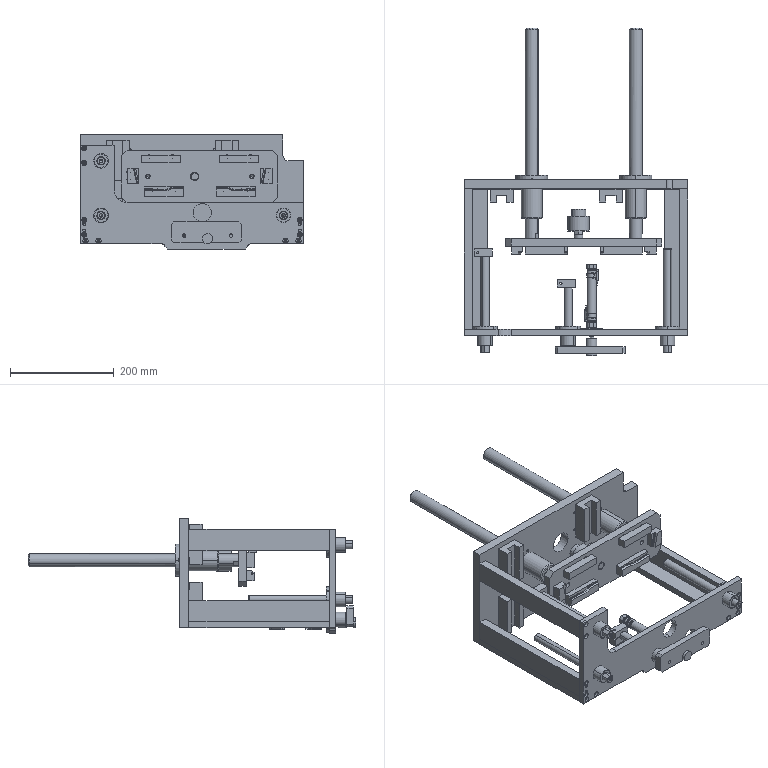Assembly | SolidWorks | mm | 39 component files | 42 solids | 1605 faces | box 430 x 630.7 x 220 mm | volume 4452531 mm3 | cylinder 737 | plane 604 | cone 208 | torus 28 | spline 24 | sphere 4 | commonest cylinder face diameters 5.5 x96 4.2 x96 10 x84 4.5 x60 8 x60 5 x52 16 x28 28 x26
Bill of materials:
FloatingJointSMCJA50-16-150 | 1 |  | Solid stepped shaft that turns about one axis. It has a large cylindrical body, a shorter cylindrical boss of smaller diameter on one end, and on the other end a short section with flat faces followed by a slim cylindrical pin with a chamfered tip.
LinearBearingMISUMILHFRD25 | 2 |  | Flanged tubular sleeve. A long cylindrical tube with a through bore ends in a thin circular flange that has four evenly spaced through holes. There is a short step where the tube meets the flange.
LinearBearingSamickLMF16UU | 4 |  | Flanged bushing with a short cylindrical hub and a central through bore. A large circular flange carries four evenly spaced through holes.
164nut1 | 1 |  | Hexagonal nut-shaped body with a round central through hole. Both faces have a chamfer, seen as curved arcs on the hex flats.
16nut | 1 |  | Thin hexagonal nut-shaped body with a large round central hole and chamfers on both faces.
16PB75UBody | 1 |  | Long cylindrical rod or tube with a polygonal wrench-flat section at each end. A small cylindrical spigot with an axial hole projects from one end, and there are shallow grooves or necks where the shaft meets each polygonal section.
16PB75URod | 1 |  | Long slender pin with a short cylindrical head at one end. The head has grooves or thin flanges around it. Near the far end the shaft steps down slightly and ends in a chamfered tip.
CS1_M_S16 | 2 |  | Compound part made of a block-like body with rounded corners and a stepped cylindrical shaft running through it. One shaft end has a flattened rectangular tip with chamfers and circumferential grooves. A thin curved strap forms a closed teardrop-shaped loop from the body.
F_PB12FA_16 | 1 |  | Flat rectangular plate with rounded corners. It has one large central through hole and two smaller through holes placed symmetrically on either side along the long axis.
Press-inFixture1 | 1 |  | Two separate, identical-looking straight rectangular bars, each with a near-square cross-section and no visible features.
Press-inFixture2 | 1 |  | Two separate elongated blocks, each with a rebate (step) running along its length. The edge of the step jogs sideways in a smooth S-curve partway along. The two bodies appear to be mirror images.
Press-inFixture3 | 1 |  | Two small separate rectangular prism blocks. One has a narrow angled groove running down one face. The other has a small notch at one top corner.
PressingMechanism-01 | 2 |  | Long, thin, flat rectangular bar with two small holes drilled into one short end face.
PressingMechanism-06 | 1 |  | Large flat rectangular plate with a rounded rectangular notch cut from one corner. It has three large round through-holes in a row and many small holes.
PressingMechanism-08 | 2 |  | Long, slender solid round rod with chamfered ends. It has a small axial hole in one end and a short flat near that end.
PressingMechanism-10 | 1 |  | Flat rectangular plate with all four corners chamfered. It has a central round hole, two smaller round holes, and many slotted holes.
PressingMechanism-11 | 2 |  | Rectangular block with a large round bore and a slit running from the bore to one side face. A smaller hole crosses the slit, drilled from the top face.
PressingMechanism-12 | 3 |  | Long rectangular bar with a deeper cross-section than unnamed part. It has drilled holes in one short end face.
PressingMechanism-13 | 1 |  | Flat L-shaped plate with a rounded inside corner and a small shallow tab along the bottom edge. It has several large round holes and many small holes.
PressingMechanism-14 | 3 |  | Slender solid round rod with chamfered ends. It has an axial hole in one end and a flat on the side near that end.
PressingMechanism-25 | 1 |  | Short, stocky solid round pin with chamfered ends. It has a small axial hole in one end and a short flat near one end.
PressingMechanism-26 | 1 |  | Thick flat bar with chamfered corners. It has two round through-holes near the ends and a U-shaped slot opening at the middle of one long edge.
PressingMechanism-31 | 1 |  | Solid stepped cylindrical pin with a large-diameter section, a reduced-diameter neck, and a short end collar.
SliderHIWINHGH20CA | 4 |  | Prismatic block of constant cross-section with a large rectangular channel running through it, giving a U-shaped profile. There are minor steps on the outer faces.
Mates:
1. concentric | LinearBearingMISUMILHFRD25-2 edge at (-70, 71, 175) dir (0, -1, 0) r 12.5 | PressingMechanism-08-2 face at (-70, -55.5, 175) dir (0, 1, 0) r 12.5
2. concentric | LinearBearingSamickLMF16UU-1 face at (191, -219, 100) dir (0, -1, 0) r 8 | PressingMechanism-14-1 face at (191, -270.389, 100) dir (0, 1, 0) r 8
3. concentric | LinearBearingSamickLMF16UU-2 face at (-160, -219, 205) dir (0, -1, 0) r 8 | PressingMechanism-14-5 face at (-160, -270.389, 205) dir (0, 1, 0) r 8
4. coincident | PressingMechanism-14-1 face at (191, -70.389, 100) dir (0, 1, 0) | PressingMechanism-14-5 face at (-160, -70.389, 205) dir (0, 1, 0)
5. coincident | SliderHIWINHGH20CA-1 face at (-106, 19.6, 245) dir (1, 0, 0) | SliderHIWINHGH20CA-6 face at (-106, 19.6, 132.5) dir (1, 0, 0)
6. distance | SliderHIWINHGH20CA-1 face at (-106, 44.6, 167.5) dir (0, 0, -1) | SliderHIWINHGH20CA-6 face at (-106, 44.6, 55) dir (0, 0, -1)
7. concentric | PressingMechanism-25-2 face at (0, -259, 61) dir (0, 1, 0) r 8 | PressingMechanism-11-4 face at (0, -144, 61) dir (0, 1, 0) r 8
8. concentric | PressingMechanism-14-7 face at (-160, -270.389, 100) dir (0, 1, 0) r 8 | LinearBearingSamickLMF16UU-5 face at (-160, -219, 100) dir (0, -1, 0) r 8
9. coincident | PressingMechanism-25-2 face at (0, -129, 61) dir (0, 1, 0) | PressingMechanism-11-4 face at (-3.5, -129, 61) dir (0, 1, 0)
10. concentric | PressingMechanism-08-2 face at (-70, -55.5, 175) dir (0, -1, 0) r 3.4 | PressingMechanism-10-1 face at (-70, -65.5, 175) dir (0, -1, 0) r 4.5
11. distance | PressingMechanism-08-2 face at (-70, -55.5, 175) dir (0, -1, 0) | PressingMechanism-10-1 face at (30, -50.5, 175) dir (0, 1, 0)
12. concentric | PressingMechanism-08-1 face at (130, -55.5, 175) dir (0, -1, 0) r 3.4 | PressingMechanism-10-1 face at (130, -65.5, 175) dir (0, -1, 0) r 4.5
13. distance | PressingMechanism-08-1 face at (130, -55.5, 175) dir (0, -1, 0) | PressingMechanism-10-1 face at (30, -50.5, 175) dir (0, 1, 0)
14. distance | FloatingJointSMCJA50-16-150-1 face at (21.632, -65.5, 177.968) dir (0, -1, 0) | PressingMechanism-10-1 face at (30, -50.5, 175) dir (0, 1, 0)
15. concentric | PressingMechanism-06-1 face at (-70, 63, 175) dir (0, 1, 0) r 20 | LinearBearingMISUMILHFRD25-2 face at (-70, 25.75, 175) dir (0, -1, 0) r 20
16. coincident | PressingMechanism-06-1 face at (-10, 63, 150) dir (0, 1, 0) | LinearBearingMISUMILHFRD25-2 face at (-70, 63, 200.25) dir (0, -1, 0)
17. distance | PressingMechanism-06-1 face at (230, 63, 45) dir (0, 0, -1) | PressingMechanism-12-2 face at (-185, -225, 57) dir (0, 0, -1)
18. coincident | PressingMechanism-06-1 face at (-200, 63, 45) dir (-1, 0, 0) | PressingMechanism-12-2 face at (-200, -90, 77) dir (-1, 0, 0)
19. coincident | PressingMechanism-06-1 face at (-10, 45, 150) dir (0, -1, 0) | PressingMechanism-12-2 face at (-185, 45, 97) dir (0, 1, 0)
20. coincident | PressingMechanism-06-1 face at (-10, 45, 150) dir (0, -1, 0) | PressingMechanism-01-4 face at (-155, 45, 45) dir (0, 1, 0)
21. coincident | PressingMechanism-01-1 face at (230, -225, 45) dir (1, 0, 0) | PressingMechanism-06-1 face at (230, 63, 45) dir (1, 0, 0)
22. coincident | PressingMechanism-01-1 face at (185, 45, 45) dir (0, 1, 0) | PressingMechanism-06-1 face at (-10, 45, 150) dir (0, -1, 0)
23. coincident | PressingMechanism-01-1 face at (207.5, -90, 45) dir (0, 0, -1) | PressingMechanism-06-1 face at (230, 63, 45) dir (0, 0, -1)
24. coincident | PressingMechanism-01-1 face at (230, -225, 45) dir (1, 0, 0) | PressingMechanism-06-1 face at (230, 63, 45) dir (1, 0, 0)
25. coincident | PressingMechanism-06-1 face at (230, 63, 45) dir (1, 0, 0) | PressingMechanism-12-1 face at (230, -90, 77) dir (1, 0, 0)
26. coincident | PressingMechanism-01-1 face at (207.5, -90, 57) dir (0, 0, 1) | PressingMechanism-12-1 face at (215, -225, 57) dir (0, 0, -1)
27. coincident | PressingMechanism-06-1 face at (-10, 45, 150) dir (0, -1, 0) | PressingMechanism-12-1 face at (215, 45, 57) dir (0, 1, 0)
28. concentric | LinearBearingMISUMILHFRD25-1 face at (130, 29.5, 175) dir (0, -1, 0) r 12.5 | PressingMechanism-08-1 face at (130, -55.5, 175) dir (0, 1, 0) r 12.5
29. coincident | PressingMechanism-06-1 face at (-10, 63, 150) dir (0, 1, 0) | LinearBearingMISUMILHFRD25-1 face at (104.751, 63, 175.213) dir (0, -1, 0)
30. coincident | PressingMechanism-12-1 face at (230, -90, 77) dir (1, 0, 0) | PressingMechanism-13-1 face at (230, -225, 45) dir (1, 0, 0)
31. coincident | PressingMechanism-12-1 face at (215, -225, 57) dir (0, -1, 0) | PressingMechanism-13-1 face at (12.5, -225, 85) dir (0, 1, 0)
32. coincident | PressingMechanism-01-1 face at (207.5, -90, 45) dir (0, 0, -1) | PressingMechanism-13-1 face at (-200, -225, 45) dir (0, 0, -1)
33. coincident | PressingMechanism-13-1 face at (12.5, -225, 85) dir (0, 1, 0) | LinearBearingSamickLMF16UU-5 face at (-160, -225, 100) dir (0, -1, 0)
34. concentric | PressingMechanism-13-1 face at (191, -225, 100) dir (0, 1, 0) r 14 | LinearBearingSamickLMF16UU-1 face at (191, -219, 100) dir (0, -1, 0) r 14
35. coincident | PressingMechanism-13-1 face at (12.5, -225, 85) dir (0, 1, 0) | LinearBearingSamickLMF16UU-1 face at (191, -225, 100) dir (0, -1, 0)
36. concentric | PressingMechanism-14-7 face at (-160, -270.389, 100) dir (0, 1, 0) r 8 | LinearBearingSamickLMF16UU-5 face at (-160, -219, 100) dir (0, -1, 0) r 14
37. concentric | PressingMechanism-14-1 face at (191, -270.389, 100) dir (0, 1, 0) r 8 | LinearBearingSamickLMF16UU-1 face at (191, -219, 100) dir (0, -1, 0) r 14
38. concentric | PressingMechanism-13-1 face at (-160, -240, 205) dir (0, 1, 0) r 14 | PressingMechanism-14-5 face at (-160, -270.389, 205) dir (0, 1, 0) r 8
39. coincident | PressingMechanism-13-1 face at (12.5, -225, 85) dir (0, 1, 0) | LinearBearingSamickLMF16UU-2 face at (-160, -225, 205) dir (0, -1, 0)
40. coincident | PressingMechanism-14-5 face at (-160, -70.389, 205) dir (0, 1, 0) | PressingMechanism-14-7 face at (-160, -70.389, 100) dir (0, 1, 0)
41. concentric | PressingMechanism-13-1 face at (35, -271, 105) dir (0, 1, 0) r 17.5 | assembly face at (35, -20.189, 105) dir (0, -1, 0) r 11
42. coincident | PressingMechanism-13-1 face at (12.5, -225, 85) dir (0, 1, 0) | assembly face at (7, -225, 90) dir (0, -1, 0)
43. parallel | PressingMechanism-13-1 face at (-200, -225, 125) dir (0, 0, 1) | assembly face at (63, -221, 124) dir (0, 0, 1)
44. coincident | PressingMechanism-10-1 face at (30, -65.5, 175) dir (0, -1, 0) | Press-inFixture1-1 face at (-45, -65.5, 208.602) dir (0, 1, 0)
45. coincident | PressingMechanism-10-1 face at (30, -65.5, 175) dir (0, -1, 0) | Press-inFixture3-1 face at (-98, -65.5, 176.102) dir (0, 1, 0)
46. coincident | PressingMechanism-10-1 face at (30, -65.5, 175) dir (0, -1, 0) | Press-inFixture2-1 face at (-39, -65.5, 146) dir (0, 1, 0)
47. coincident | PressingMechanism-06-1 face at (-10, 45, 150) dir (0, -1, 0) | SliderHIWINHGH20CA-1 face at (-106, 45, 181) dir (0, 1, 0)
48. coincident | PressingMechanism-12-2 face at (-185, -225, 57) dir (0, 0, -1) | PressingMechanism-01-4 face at (-177.5, -90, 57) dir (0, 0, 1)
49. coincident | PressingMechanism-12-2 face at (-200, -90, 77) dir (-1, 0, 0) | PressingMechanism-01-4 face at (-200, 45, 45) dir (-1, 0, 0)
50. coincident | PressingMechanism-26-1 face at (45, -259, 62.5) dir (0, 1, 0) | PressingMechanism-31-1 face at (45, -259, 55) dir (0, -1, 0)
51. concentric | PressingMechanism-25-2 face at (0, -259, 61) dir (0, 1, 0) r 8 | PressingMechanism-26-1 face at (0, -259, 61) dir (0, 1, 0) r 3.3
52. distance | SliderHIWINHGH20CA-5 face at (104, 44.6, 245) dir (0, 0, 1) | PressingMechanism-06-1 face at (230, 63, 255) dir (0, 0, 1)
53. coincident | SliderHIWINHGH20CA-7 face at (104, 19.6, 132.5) dir (1, 0, 0) | SliderHIWINHGH20CA-5 face at (104, 19.6, 245) dir (1, 0, 0)
54. distance | SliderHIWINHGH20CA-1 face at (-150, 44.6, 245) dir (-1, 0, 0) | PressingMechanism-06-1 face at (-200, 63, 45) dir (-1, 0, 0)
55. concentric | PressingMechanism-13-1 face at (0, -192, 61) dir (0, -1, 0) r 14 | LinearBearingSamickLMF16UU-4 face at (0, -219, 61) dir (0, -1, 0) r 14
56. coincident | PressingMechanism-13-1 face at (12.5, -225, 85) dir (0, 1, 0) | LinearBearingSamickLMF16UU-4 face at (0, -225, 61) dir (0, -1, 0)
57. concentric | LinearBearingSamickLMF16UU-4 face at (0, -219, 61) dir (0, -1, 0) r 8 | PressingMechanism-25-2 face at (0, -259, 61) dir (0, 1, 0) r 8
58. coincident | PressingMechanism-25-2 face at (0, -259, 61) dir (0, -1, 0) | PressingMechanism-26-1 face at (45, -259, 62.5) dir (0, 1, 0)
59. coincident | PressingMechanism-06-1 face at (-10, 45, 150) dir (0, -1, 0) | PressingMechanism-12-3 face at (-185, 45, 235) dir (0, 1, 0)
60. coincident | PressingMechanism-13-1 face at (-200, -225, 45) dir (-1, 0, 0) | PressingMechanism-12-3 face at (-200, -90, 215) dir (-1, 0, 0)
61. distance | PressingMechanism-12-3 face at (-185, -225, 235) dir (0, 0, 1) | PressingMechanism-13-1 face at (-200, -364.769, 235) dir (0, 0, 1)
62. concentric | PressingMechanism-06-1 face at (130, 63, 175) dir (0, 1, 0) r 20 | LinearBearingMISUMILHFRD25-1 face at (130, 25.75, 175) dir (0, -1, 0) r 20
63. concentric | PressingMechanism-13-1 face at (-160, -225, 100) dir (0, 1, 0) r 14 | LinearBearingSamickLMF16UU-5 face at (-160, -219, 100) dir (0, -1, 0) r 14
64. concentric | PressingMechanism-13-1 face at (45, -225, 55) dir (0, 1, 0) r 9 | PB_16x75_S_U_FA_M_2_0-1/16PB75UBody-1 face at (45, -222.5, 55) dir (0, -1, 0) r 5
65. coincident | PressingMechanism-13-1 face at (12.5, -225, 85) dir (0, 1, 0) | PB_16x75_S_U_FA_M_2_0-1/F_PB12FA_16-1 face at (26, -225, 63) dir (0, -1, 0)
66. parallel | PressingMechanism-13-1 face at (-37.5, -237, 35) dir (0, 0, -1) | PB_16x75_S_U_FA_M_2_0-1/F_PB12FA_16-1 face at (64, -222.5, 65) dir (0, 0, 1)
67. concentric | PressingMechanism-31-1 face at (45, -243, 55) dir (0, -1, 0) r 10 | PB_16x75_S_U_FA_M_2_0-1/16PB75URod-1 face at (45, -115.14, 55) dir (0, -1, 0) r 2.5
68. concentric | PressingMechanism-14-5 face at (-160, -270.389, 205) dir (0, 1, 0) r 8 | PressingMechanism-11-5 face at (-160, -85.389, 205) dir (0, 1, 0) r 8
69. coincident | PressingMechanism-14-5 face at (-160, -70.389, 205) dir (0, 1, 0) | PressingMechanism-11-5 face at (-163.5, -70.389, 205) dir (0, 1, 0)
70. coincident | 16PB75UBody-1 axis at (-100.7, 0, 0) dir (1, 0, 0) | 16PB75URod-1 axis at (-120.7, 0, 0) dir (1, 0, 0)
71. coincident | 16PB75UBody-1 axis at (-100.7, 0, 0) dir (1, 0, 0) | 16PB75URod-1 axis at (-120.7, 0, 0) dir (1, 0, 0)
72. coincident | 16PB75UBody-1 axis at (-100.7, 0, 0) dir (1, 0, 0) | 16PB75URod-1 axis at (-120.7, 0, 0) dir (1, 0, 0)
73. angle | 16PB75URod-1 plane at (-39.8, 0, 0) dir (0, 0, -1) | 16PB75UBody-1 plane at (-19.8, 0, 0) dir (0, 0, -1)